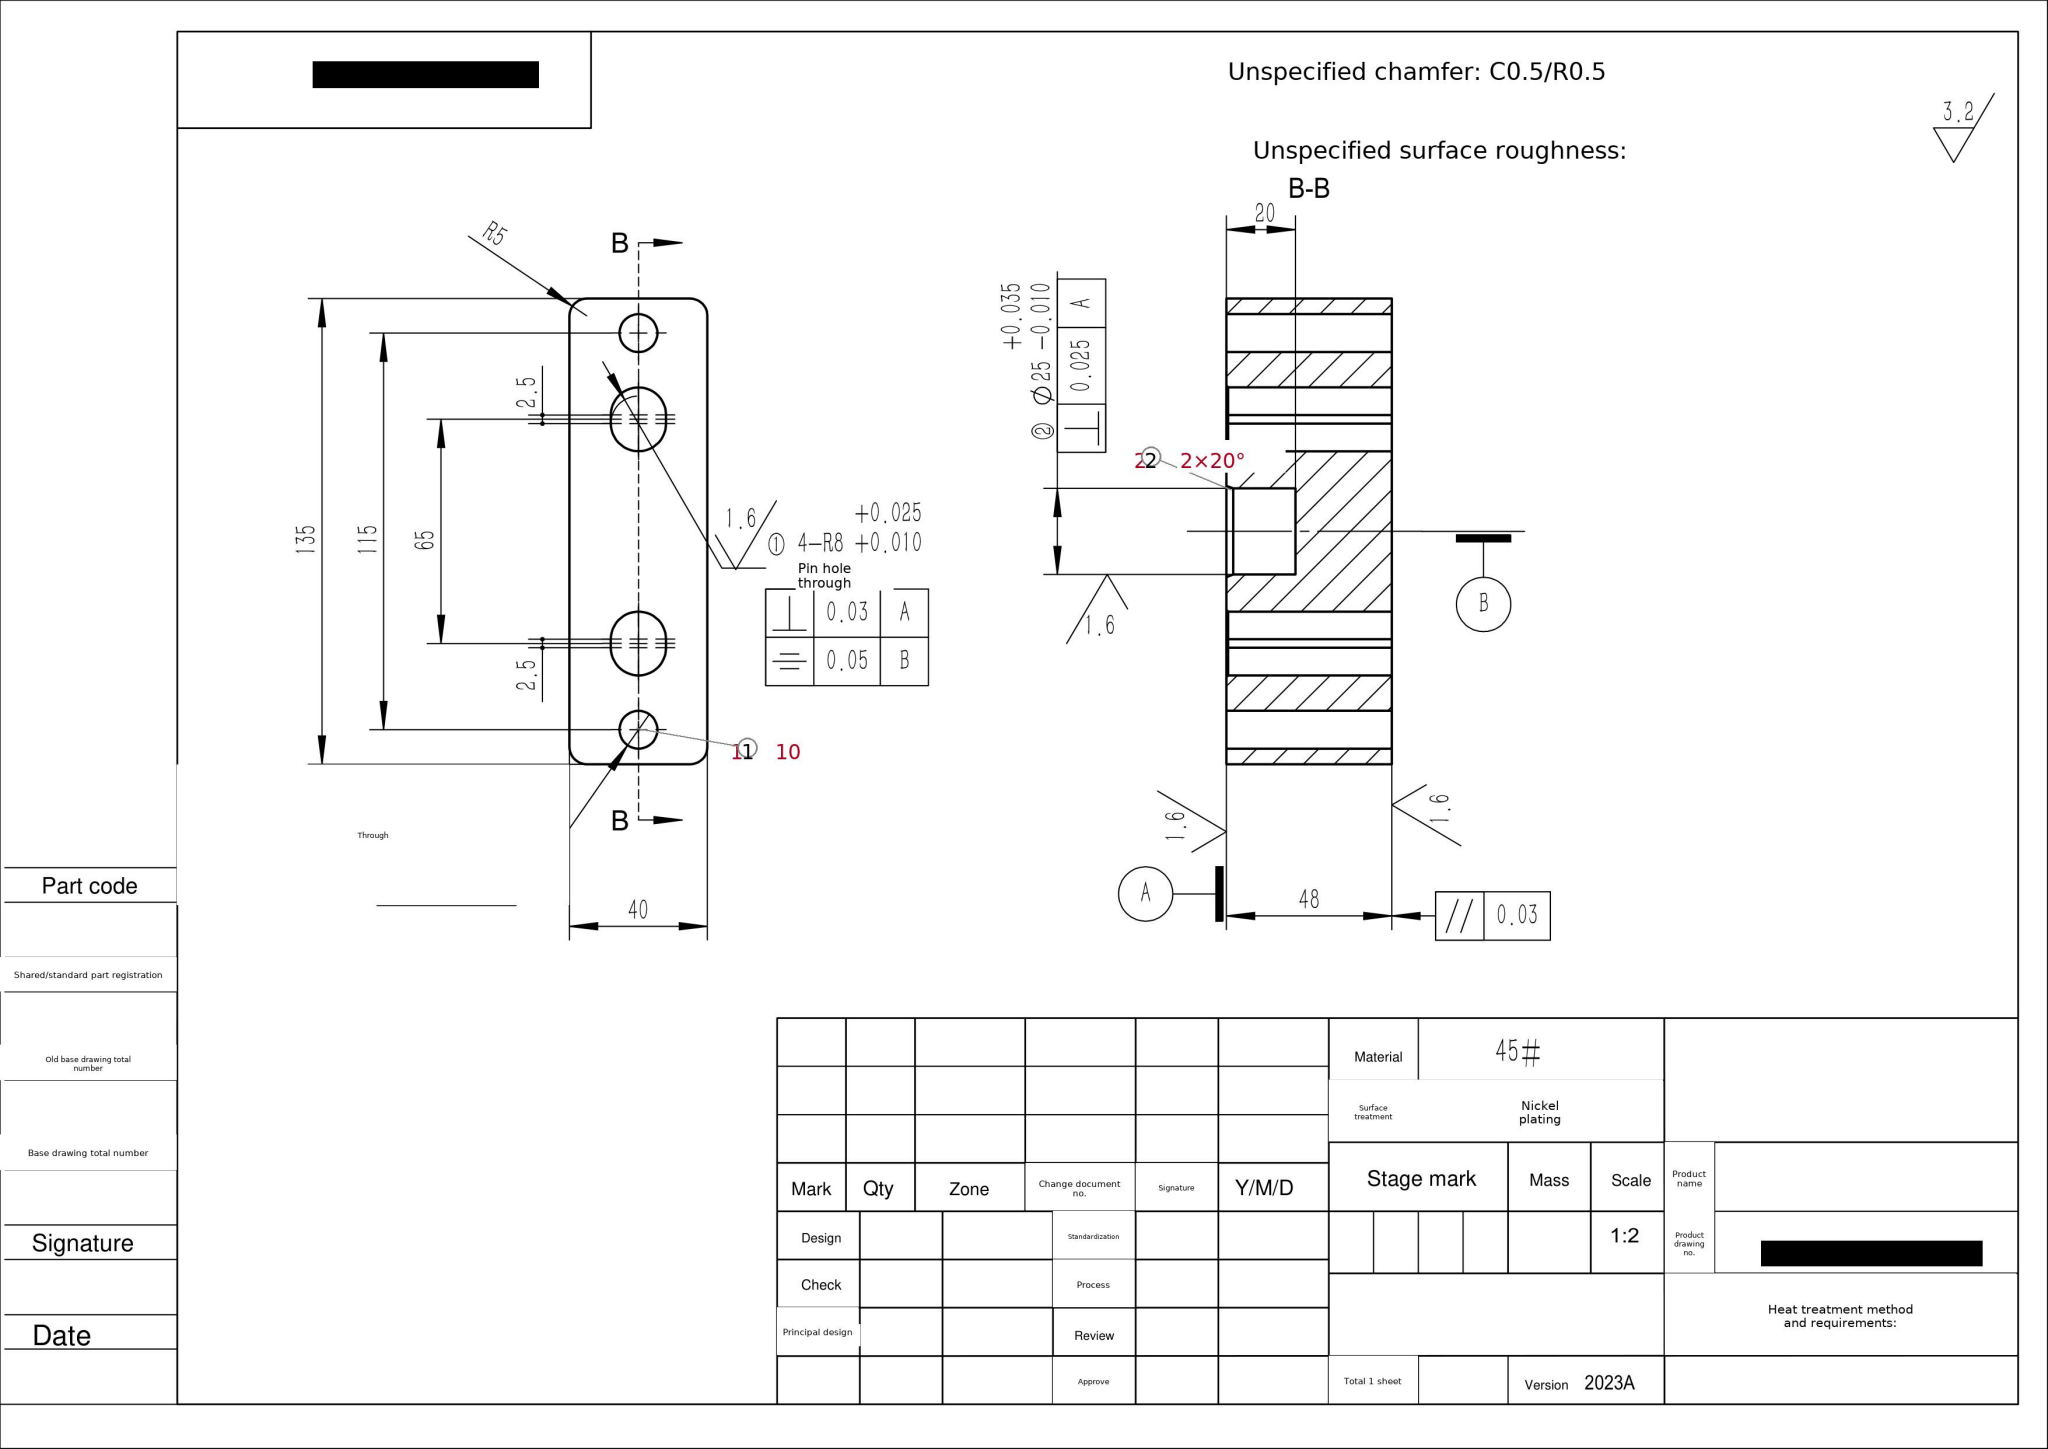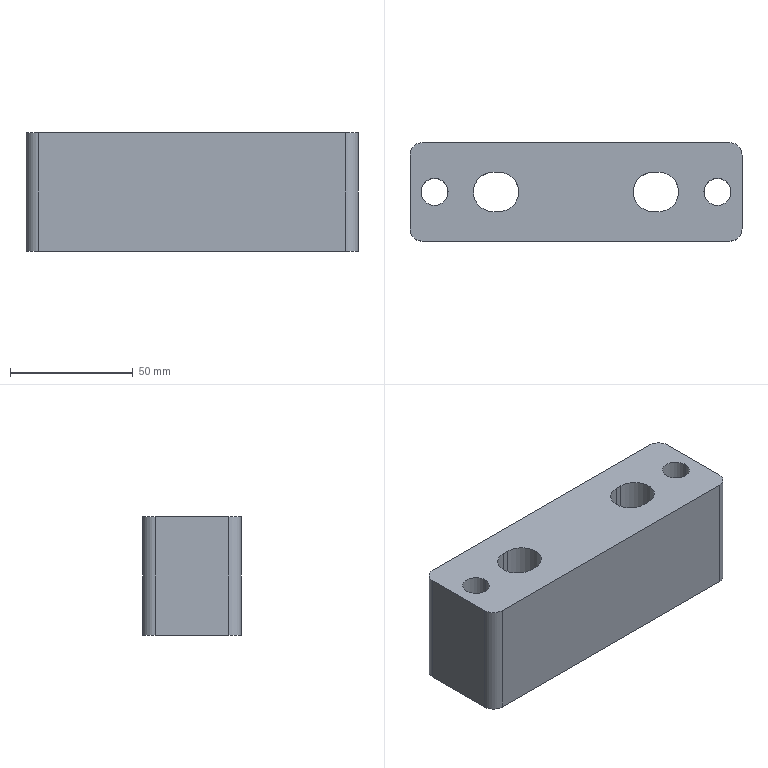Part | SolidWorks | mm | material 45# | 1 solid | 39 faces | box 135 x 40 x 48 mm | volume 216015 mm3 | cylinder 16 | plane 15 | cone 8 | commonest cylinder face diameters 16 x6 11 x4 10 x4 25 x2
build123d program:
from build123d import *

# Parameters (mm, degrees)
SKETCH1_W           = 135
SKETCH1_H           = 40
BOSS_EXTRUDE1_DEPTH = 48
SKETCH2_R           = 5.5
CUT_EXTRUDE1_DEPTH  = 86.207
SKETCH7_R           = 12.5
CUT_EXTRUDE5_DEPTH  = 20
CHAMFER4_SIZE       = 2
CHAMFER4_SIZE2      = 0.7279
CUT_EXTRUDE6_DEPTH  = 86.207
FILLET1_R           = 5
CHAMFER8_SIZE       = 0.5


with BuildPart() as part:
    # Sketch1 → Boss-Extrude1 (new body)
    with BuildSketch(Plane.XY):
        Rectangle(SKETCH1_W, SKETCH1_H)
    extrude(amount=BOSS_EXTRUDE1_DEPTH)

    # Sketch2 → Cut-Extrude1 (cut, through all)
    with BuildSketch(Plane.XY.offset(48)):
        with Locations((-57.5, 0)):
            Circle(SKETCH2_R)
        with Locations((57.5, 0)):
            Circle(SKETCH2_R)
    extrude(amount=-CUT_EXTRUDE1_DEPTH, mode=Mode.SUBTRACT)

    # Sketch7 → Cut-Extrude5 (cut)
    with BuildSketch(Plane(origin=(0, 0, 0), x_dir=(-1, 0, 0), z_dir=(0, 0, -1))):
        Circle(SKETCH7_R)
    extrude(amount=-CUT_EXTRUDE5_DEPTH, mode=Mode.SUBTRACT)

    # Chamfer4
    chamfer4_edges = [part.edges().sort_by_distance(p)[0] for p in [
        (12.5, 0, 0),
    ]]
    chamfer4_side = [part.faces().sort_by_distance(p)[0] for p in [
        (12.5, 0, 10),
    ]]
    chamfer(chamfer4_edges, length=CHAMFER4_SIZE, length2=CHAMFER4_SIZE2, reference=chamfer4_side[0])

    # Sketch8 → Cut-Extrude6 (cut, through all)
    with BuildSketch(Plane(origin=(0, 0, 0), x_dir=(-1, 0, 0), z_dir=(0, 0, -1))):
        with BuildLine():
            Line((33.75, -8), (31.25, -8))
            ThreePointArc((31.25, -8), (23.25, 0), (31.25, 8))
            Line((31.25, 8), (33.75, 8))
            ThreePointArc((33.75, 8), (41.75, 0), (33.75, -8))
        make_face()
        with BuildLine():
            Line((-31.25, -8), (-33.75, -8))
            ThreePointArc((-33.75, -8), (-41.75, 0), (-33.75, 8))
            Line((-33.75, 8), (-31.25, 8))
            ThreePointArc((-31.25, 8), (-23.25, 0), (-31.25, -8))
        make_face()
    extrude(amount=-CUT_EXTRUDE6_DEPTH, mode=Mode.SUBTRACT)

    # Fillet1
    fillet1_edges = [part.edges().sort_by_distance(p)[0] for p in [
        (67.5, -20, 24),
        (-67.5, -20, 24),
        (-67.5, 20, 24),
        (67.5, 20, 24),
    ]]
    fillet(fillet1_edges, radius=FILLET1_R)

    # Chamfer8
    chamfer8_edges = [part.edges().sort_by_distance(p)[0] for p in [
        (-41.75, 0, 0),
        (-32.5, 8, 0),
        (-23.25, 0, 0),
        (-32.5, -8, 0),
        (23.25, 0, 0),
        (32.5, 8, 0),
        (41.75, 0, 0),
        (32.5, -8, 0),
    ]]
    chamfer(chamfer8_edges, length=CHAMFER8_SIZE)


solid = part.part